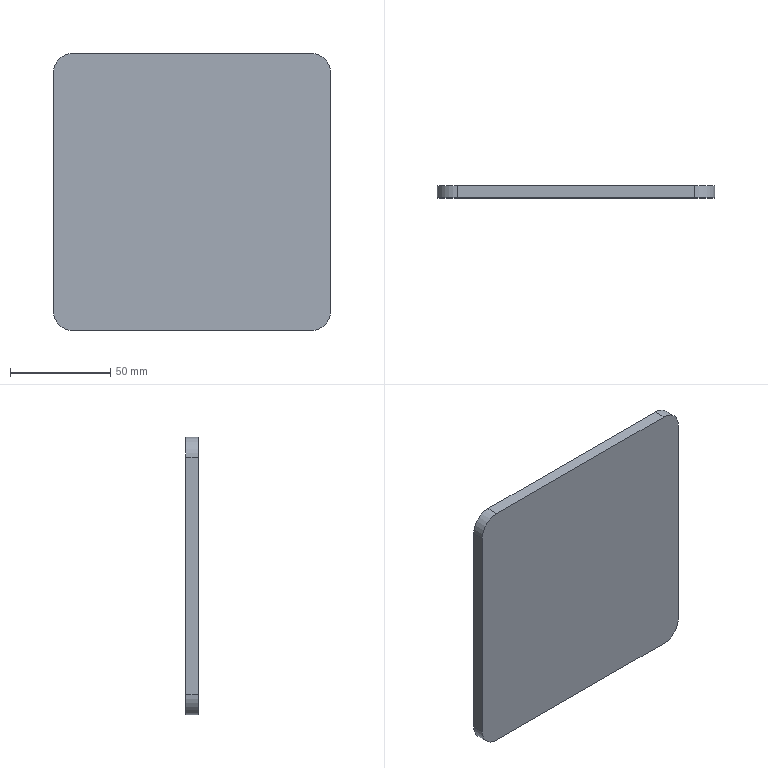Component | SolidWorks | Block-1 | 1 solid | 10 faces | box 138 x 6 x 138 mm | volume 113749 mm3 | plane 6 | cylinder 4 | commonest cylinder face diameters 20 x4 | material Plain Carbon Steel
STEP:
#1=CARTESIAN_POINT('',(170.228,107.729,218.897));
#2=VERTEX_POINT('',#1);
#3=CARTESIAN_POINT('',(170.622,107.729,219.29));
#4=VERTEX_POINT('',#3);
#5=CARTESIAN_POINT('',(170.622,107.729,218.897));
#6=DIRECTION('',(0.,1.,0.));
#7=DIRECTION('',(0.,0.,1.));
#8=AXIS2_PLACEMENT_3D('',#5,#6,#7);
#9=CIRCLE('',#8,0.3937);
#10=EDGE_CURVE('',#2,#4,#9,.T.);
#11=ORIENTED_EDGE('',*,*,#10,.F.);
#12=CARTESIAN_POINT('',(170.228,107.493,218.897));
#13=VERTEX_POINT('',#12);
#14=CARTESIAN_POINT('',(170.228,107.493,218.897));
#15=DIRECTION('',(0.,1.,0.));
#16=VECTOR('',#15,39.37);
#17=LINE('',#14,#16);
#18=EDGE_CURVE('',#13,#2,#17,.T.);
#19=ORIENTED_EDGE('',*,*,#18,.F.);
#20=CARTESIAN_POINT('',(170.622,107.493,219.29));
#21=VERTEX_POINT('',#20);
#22=CARTESIAN_POINT('',(170.622,107.493,218.897));
#23=DIRECTION('',(0.,1.,0.));
#24=DIRECTION('',(0.,0.,1.));
#25=AXIS2_PLACEMENT_3D('',#22,#23,#24);
#26=CIRCLE('',#25,0.3937);
#27=EDGE_CURVE('',#13,#21,#26,.T.);
#28=ORIENTED_EDGE('',*,*,#27,.T.);
#29=CARTESIAN_POINT('',(170.622,107.493,219.29));
#30=DIRECTION('',(0.,1.,0.));
#31=VECTOR('',#30,39.37);
#32=LINE('',#29,#31);
#33=EDGE_CURVE('',#21,#4,#32,.T.);
#34=ORIENTED_EDGE('',*,*,#33,.T.);
#35=EDGE_LOOP('',(#11,#19,#28,#34));
#36=FACE_OUTER_BOUND('',#35,.T.);
#37=CARTESIAN_POINT('',(170.622,107.493,218.897));
#38=DIRECTION('',(0.,1.,0.));
#39=DIRECTION('',(0.,0.,1.));
#40=AXIS2_PLACEMENT_3D('',#37,#38,#39);
#41=CYLINDRICAL_SURFACE('',#40,0.3937);
#42=ADVANCED_FACE('',(#36),#41,.T.);
#43=CARTESIAN_POINT('',(170.228,107.729,214.251));
#44=VERTEX_POINT('',#43);
#45=CARTESIAN_POINT('',(170.228,107.729,214.251));
#46=DIRECTION('',(0.,0.,1.));
#47=VECTOR('',#46,39.37);
#48=LINE('',#45,#47);
#49=EDGE_CURVE('',#44,#2,#48,.T.);
#50=ORIENTED_EDGE('',*,*,#49,.F.);
#51=CARTESIAN_POINT('',(170.228,107.493,214.251));
#52=VERTEX_POINT('',#51);
#53=CARTESIAN_POINT('',(170.228,107.493,214.251));
#54=DIRECTION('',(0.,1.,0.));
#55=VECTOR('',#54,39.37);
#56=LINE('',#53,#55);
#57=EDGE_CURVE('',#52,#44,#56,.T.);
#58=ORIENTED_EDGE('',*,*,#57,.F.);
#59=CARTESIAN_POINT('',(170.228,107.493,214.251));
#60=DIRECTION('',(0.,0.,1.));
#61=VECTOR('',#60,39.37);
#62=LINE('',#59,#61);
#63=EDGE_CURVE('',#52,#13,#62,.T.);
#64=ORIENTED_EDGE('',*,*,#63,.T.);
#65=ORIENTED_EDGE('',*,*,#18,.T.);
#66=EDGE_LOOP('',(#50,#58,#64,#65));
#67=FACE_OUTER_BOUND('',#66,.T.);
#68=CARTESIAN_POINT('',(170.228,107.493,214.251));
#69=DIRECTION('',(-1.,0.,0.));
#70=DIRECTION('',(0.,0.,1.));
#71=AXIS2_PLACEMENT_3D('',#68,#69,#70);
#72=PLANE('',#71);
#73=ADVANCED_FACE('',(#67),#72,.T.);
#74=CARTESIAN_POINT('',(170.622,107.729,213.857));
#75=VERTEX_POINT('',#74);
#76=CARTESIAN_POINT('',(170.622,107.729,214.251));
#77=DIRECTION('',(0.,1.,0.));
#78=DIRECTION('',(0.,0.,1.));
#79=AXIS2_PLACEMENT_3D('',#76,#77,#78);
#80=CIRCLE('',#79,0.3937);
#81=EDGE_CURVE('',#75,#44,#80,.T.);
#82=ORIENTED_EDGE('',*,*,#81,.F.);
#83=CARTESIAN_POINT('',(170.622,107.493,213.857));
#84=VERTEX_POINT('',#83);
#85=CARTESIAN_POINT('',(170.622,107.493,213.857));
#86=DIRECTION('',(0.,1.,0.));
#87=VECTOR('',#86,39.37);
#88=LINE('',#85,#87);
#89=EDGE_CURVE('',#84,#75,#88,.T.);
#90=ORIENTED_EDGE('',*,*,#89,.F.);
#91=CARTESIAN_POINT('',(170.622,107.493,214.251));
#92=DIRECTION('',(0.,1.,0.));
#93=DIRECTION('',(0.,0.,1.));
#94=AXIS2_PLACEMENT_3D('',#91,#92,#93);
#95=CIRCLE('',#94,0.3937);
#96=EDGE_CURVE('',#84,#52,#95,.T.);
#97=ORIENTED_EDGE('',*,*,#96,.T.);
#98=ORIENTED_EDGE('',*,*,#57,.T.);
#99=EDGE_LOOP('',(#82,#90,#97,#98));
#100=FACE_OUTER_BOUND('',#99,.T.);
#101=CARTESIAN_POINT('',(170.622,107.493,214.251));
#102=DIRECTION('',(0.,1.,0.));
#103=DIRECTION('',(0.,0.,1.));
#104=AXIS2_PLACEMENT_3D('',#101,#102,#103);
#105=CYLINDRICAL_SURFACE('',#104,0.3937);
#106=ADVANCED_FACE('',(#100),#105,.T.);
#107=CARTESIAN_POINT('',(175.268,107.729,213.857));
#108=VERTEX_POINT('',#107);
#109=CARTESIAN_POINT('',(170.622,107.729,213.857));
#110=DIRECTION('',(-1.,0.,0.));
#111=VECTOR('',#110,39.37);
#112=LINE('',#109,#111);
#113=EDGE_CURVE('',#108,#75,#112,.T.);
#114=ORIENTED_EDGE('',*,*,#113,.F.);
#115=CARTESIAN_POINT('',(175.268,107.493,213.857));
#116=VERTEX_POINT('',#115);
#117=CARTESIAN_POINT('',(175.268,107.493,213.857));
#118=DIRECTION('',(0.,1.,0.));
#119=VECTOR('',#118,39.37);
#120=LINE('',#117,#119);
#121=EDGE_CURVE('',#116,#108,#120,.T.);
#122=ORIENTED_EDGE('',*,*,#121,.F.);
#123=CARTESIAN_POINT('',(170.622,107.493,213.857));
#124=DIRECTION('',(-1.,0.,0.));
#125=VECTOR('',#124,39.37);
#126=LINE('',#123,#125);
#127=EDGE_CURVE('',#116,#84,#126,.T.);
#128=ORIENTED_EDGE('',*,*,#127,.T.);
#129=ORIENTED_EDGE('',*,*,#89,.T.);
#130=EDGE_LOOP('',(#114,#122,#128,#129));
#131=FACE_OUTER_BOUND('',#130,.T.);
#132=CARTESIAN_POINT('',(170.622,107.493,213.857));
#133=DIRECTION('',(0.,0.,-1.));
#134=DIRECTION('',(-1.,0.,0.));
#135=AXIS2_PLACEMENT_3D('',#132,#133,#134);
#136=PLANE('',#135);
#137=ADVANCED_FACE('',(#131),#136,.T.);
#138=CARTESIAN_POINT('',(175.661,107.729,214.251));
#139=VERTEX_POINT('',#138);
#140=CARTESIAN_POINT('',(175.268,107.729,214.251));
#141=DIRECTION('',(0.,1.,0.));
#142=DIRECTION('',(0.,0.,-1.));
#143=AXIS2_PLACEMENT_3D('',#140,#141,#142);
#144=CIRCLE('',#143,0.3937);
#145=EDGE_CURVE('',#139,#108,#144,.T.);
#146=ORIENTED_EDGE('',*,*,#145,.F.);
#147=CARTESIAN_POINT('',(175.661,107.493,214.251));
#148=VERTEX_POINT('',#147);
#149=CARTESIAN_POINT('',(175.661,107.493,214.251));
#150=DIRECTION('',(0.,1.,0.));
#151=VECTOR('',#150,39.37);
#152=LINE('',#149,#151);
#153=EDGE_CURVE('',#148,#139,#152,.T.);
#154=ORIENTED_EDGE('',*,*,#153,.F.);
#155=CARTESIAN_POINT('',(175.268,107.493,214.251));
#156=DIRECTION('',(0.,1.,0.));
#157=DIRECTION('',(0.,0.,-1.));
#158=AXIS2_PLACEMENT_3D('',#155,#156,#157);
#159=CIRCLE('',#158,0.3937);
#160=EDGE_CURVE('',#148,#116,#159,.T.);
#161=ORIENTED_EDGE('',*,*,#160,.T.);
#162=ORIENTED_EDGE('',*,*,#121,.T.);
#163=EDGE_LOOP('',(#146,#154,#161,#162));
#164=FACE_OUTER_BOUND('',#163,.T.);
#165=CARTESIAN_POINT('',(175.268,107.493,214.251));
#166=DIRECTION('',(0.,1.,0.));
#167=DIRECTION('',(0.,0.,1.));
#168=AXIS2_PLACEMENT_3D('',#165,#166,#167);
#169=CYLINDRICAL_SURFACE('',#168,0.3937);
#170=ADVANCED_FACE('',(#164),#169,.T.);
#171=CARTESIAN_POINT('',(175.661,107.729,218.897));
#172=VERTEX_POINT('',#171);
#173=CARTESIAN_POINT('',(175.661,107.729,214.251));
#174=DIRECTION('',(0.,0.,-1.));
#175=VECTOR('',#174,39.37);
#176=LINE('',#173,#175);
#177=EDGE_CURVE('',#172,#139,#176,.T.);
#178=ORIENTED_EDGE('',*,*,#177,.F.);
#179=CARTESIAN_POINT('',(175.661,107.493,218.897));
#180=VERTEX_POINT('',#179);
#181=CARTESIAN_POINT('',(175.661,107.493,218.897));
#182=DIRECTION('',(0.,1.,0.));
#183=VECTOR('',#182,39.37);
#184=LINE('',#181,#183);
#185=EDGE_CURVE('',#180,#172,#184,.T.);
#186=ORIENTED_EDGE('',*,*,#185,.F.);
#187=CARTESIAN_POINT('',(175.661,107.493,214.251));
#188=DIRECTION('',(0.,0.,-1.));
#189=VECTOR('',#188,39.37);
#190=LINE('',#187,#189);
#191=EDGE_CURVE('',#180,#148,#190,.T.);
#192=ORIENTED_EDGE('',*,*,#191,.T.);
#193=ORIENTED_EDGE('',*,*,#153,.T.);
#194=EDGE_LOOP('',(#178,#186,#192,#193));
#195=FACE_OUTER_BOUND('',#194,.T.);
#196=CARTESIAN_POINT('',(175.661,107.493,214.251));
#197=DIRECTION('',(1.,0.,0.));
#198=DIRECTION('',(0.,0.,-1.));
#199=AXIS2_PLACEMENT_3D('',#196,#197,#198);
#200=PLANE('',#199);
#201=ADVANCED_FACE('',(#195),#200,.T.);
#202=CARTESIAN_POINT('',(175.268,107.729,219.29));
#203=VERTEX_POINT('',#202);
#204=CARTESIAN_POINT('',(175.268,107.729,218.897));
#205=DIRECTION('',(0.,1.,0.));
#206=DIRECTION('',(0.,0.,1.));
#207=AXIS2_PLACEMENT_3D('',#204,#205,#206);
#208=CIRCLE('',#207,0.3937);
#209=EDGE_CURVE('',#203,#172,#208,.T.);
#210=ORIENTED_EDGE('',*,*,#209,.F.);
#211=CARTESIAN_POINT('',(175.268,107.493,219.29));
#212=VERTEX_POINT('',#211);
#213=CARTESIAN_POINT('',(175.268,107.493,219.29));
#214=DIRECTION('',(0.,1.,0.));
#215=VECTOR('',#214,39.37);
#216=LINE('',#213,#215);
#217=EDGE_CURVE('',#212,#203,#216,.T.);
#218=ORIENTED_EDGE('',*,*,#217,.F.);
#219=CARTESIAN_POINT('',(175.268,107.493,218.897));
#220=DIRECTION('',(0.,1.,0.));
#221=DIRECTION('',(0.,0.,1.));
#222=AXIS2_PLACEMENT_3D('',#219,#220,#221);
#223=CIRCLE('',#222,0.3937);
#224=EDGE_CURVE('',#212,#180,#223,.T.);
#225=ORIENTED_EDGE('',*,*,#224,.T.);
#226=ORIENTED_EDGE('',*,*,#185,.T.);
#227=EDGE_LOOP('',(#210,#218,#225,#226));
#228=FACE_OUTER_BOUND('',#227,.T.);
#229=CARTESIAN_POINT('',(175.268,107.493,218.897));
#230=DIRECTION('',(0.,1.,0.));
#231=DIRECTION('',(0.,0.,1.));
#232=AXIS2_PLACEMENT_3D('',#229,#230,#231);
#233=CYLINDRICAL_SURFACE('',#232,0.3937);
#234=ADVANCED_FACE('',(#228),#233,.T.);
#235=CARTESIAN_POINT('',(170.622,107.729,219.29));
#236=DIRECTION('',(1.,0.,0.));
#237=VECTOR('',#236,39.37);
#238=LINE('',#235,#237);
#239=EDGE_CURVE('',#4,#203,#238,.T.);
#240=ORIENTED_EDGE('',*,*,#239,.F.);
#241=ORIENTED_EDGE('',*,*,#33,.F.);
#242=CARTESIAN_POINT('',(170.622,107.493,219.29));
#243=DIRECTION('',(1.,0.,0.));
#244=VECTOR('',#243,39.37);
#245=LINE('',#242,#244);
#246=EDGE_CURVE('',#21,#212,#245,.T.);
#247=ORIENTED_EDGE('',*,*,#246,.T.);
#248=ORIENTED_EDGE('',*,*,#217,.T.);
#249=EDGE_LOOP('',(#240,#241,#247,#248));
#250=FACE_OUTER_BOUND('',#249,.T.);
#251=CARTESIAN_POINT('',(170.622,107.493,219.29));
#252=DIRECTION('',(0.,0.,1.));
#253=DIRECTION('',(1.,0.,0.));
#254=AXIS2_PLACEMENT_3D('',#251,#252,#253);
#255=PLANE('',#254);
#256=ADVANCED_FACE('',(#250),#255,.T.);
#257=ORIENTED_EDGE('',*,*,#27,.F.);
#258=ORIENTED_EDGE('',*,*,#63,.F.);
#259=ORIENTED_EDGE('',*,*,#96,.F.);
#260=ORIENTED_EDGE('',*,*,#127,.F.);
#261=ORIENTED_EDGE('',*,*,#160,.F.);
#262=ORIENTED_EDGE('',*,*,#191,.F.);
#263=ORIENTED_EDGE('',*,*,#224,.F.);
#264=ORIENTED_EDGE('',*,*,#246,.F.);
#265=EDGE_LOOP('',(#257,#258,#259,#260,#261,#262,#263,#264));
#266=FACE_OUTER_BOUND('',#265,.T.);
#267=CARTESIAN_POINT('',(170.622,107.493,218.897));
#268=DIRECTION('',(0.,1.,0.));
#269=DIRECTION('',(0.,0.,1.));
#270=AXIS2_PLACEMENT_3D('',#267,#268,#269);
#271=PLANE('',#270);
#272=ADVANCED_FACE('',(#266),#271,.F.);
#273=ORIENTED_EDGE('',*,*,#10,.T.);
#274=ORIENTED_EDGE('',*,*,#239,.T.);
#275=ORIENTED_EDGE('',*,*,#209,.T.);
#276=ORIENTED_EDGE('',*,*,#177,.T.);
#277=ORIENTED_EDGE('',*,*,#145,.T.);
#278=ORIENTED_EDGE('',*,*,#113,.T.);
#279=ORIENTED_EDGE('',*,*,#81,.T.);
#280=ORIENTED_EDGE('',*,*,#49,.T.);
#281=EDGE_LOOP('',(#273,#274,#275,#276,#277,#278,#279,#280));
#282=FACE_OUTER_BOUND('',#281,.T.);
#283=CARTESIAN_POINT('',(170.622,107.729,218.897));
#284=DIRECTION('',(0.,1.,0.));
#285=DIRECTION('',(0.,0.,1.));
#286=AXIS2_PLACEMENT_3D('',#283,#284,#285);
#287=PLANE('',#286);
#288=ADVANCED_FACE('',(#282),#287,.T.);
#289=CLOSED_SHELL('',(#42,#73,#106,#137,#170,#201,#234,#256,#272,#288));
#290=MANIFOLD_SOLID_BREP('',#289);
#291=CARTESIAN_POINT('',(0.,0.,0.));
#292=DIRECTION('',(0.,0.,1.));
#293=DIRECTION('',(1.,0.,0.));
#294=AXIS2_PLACEMENT_3D('',#291,#292,#293);
#295=(LENGTH_UNIT()NAMED_UNIT(*)SI_UNIT($,.METRE.));
#296=LENGTH_MEASURE_WITH_UNIT(LENGTH_MEASURE(0.0254),#295);
#297=DIMENSIONAL_EXPONENTS(1.,0.,0.,0.,0.,0.,0.);
#298=(CONVERSION_BASED_UNIT('',#296)LENGTH_UNIT()NAMED_UNIT(#297));
#299=UNCERTAINTY_MEASURE_WITH_UNIT(LENGTH_MEASURE(0.00001),#298,'','');
#300=(NAMED_UNIT(*)PLANE_ANGLE_UNIT()SI_UNIT($,.RADIAN.));
#301=(NAMED_UNIT(*)SI_UNIT($,.STERADIAN.)SOLID_ANGLE_UNIT());
#302=(GEOMETRIC_REPRESENTATION_CONTEXT(3)GLOBAL_UNCERTAINTY_ASSIGNED_CONTEXT((#299))GLOBAL_UNIT_ASSIGNED_CONTEXT((#298,#300,#301))REPRESENTATION_CONTEXT('',''));
#303=ADVANCED_BREP_SHAPE_REPRESENTATION('',(#290,#294),#302);
#304=COLOUR_RGB('',0.7922,0.8196,0.9333);
#305=FILL_AREA_STYLE_COLOUR('',#304);
#306=FILL_AREA_STYLE('',(#305));
#307=SURFACE_STYLE_FILL_AREA(#306);
#308=SURFACE_SIDE_STYLE('',(#307));
#309=SURFACE_STYLE_USAGE(.BOTH.,#308);
#310=PRESENTATION_STYLE_ASSIGNMENT((#309));
#311=STYLED_ITEM('',(#310),#290);
#312=(LENGTH_UNIT()NAMED_UNIT(*)SI_UNIT($,.METRE.));
#313=LENGTH_MEASURE_WITH_UNIT(LENGTH_MEASURE(0.0254),#312);
#314=DIMENSIONAL_EXPONENTS(1.,0.,0.,0.,0.,0.,0.);
#315=(CONVERSION_BASED_UNIT('',#313)LENGTH_UNIT()NAMED_UNIT(#314));
#316=UNCERTAINTY_MEASURE_WITH_UNIT(LENGTH_MEASURE(0.00001),#315,'','');
#317=(NAMED_UNIT(*)PLANE_ANGLE_UNIT()SI_UNIT($,.RADIAN.));
#318=(NAMED_UNIT(*)SI_UNIT($,.STERADIAN.)SOLID_ANGLE_UNIT());
#319=(GEOMETRIC_REPRESENTATION_CONTEXT(3)GLOBAL_UNCERTAINTY_ASSIGNED_CONTEXT((#316))GLOBAL_UNIT_ASSIGNED_CONTEXT((#315,#317,#318))REPRESENTATION_CONTEXT('',''));
#320=MECHANICAL_DESIGN_GEOMETRIC_PRESENTATION_REPRESENTATION('',(#311),#319);
#321=PRESENTATION_LAYER_ASSIGNMENT('','',(#311));